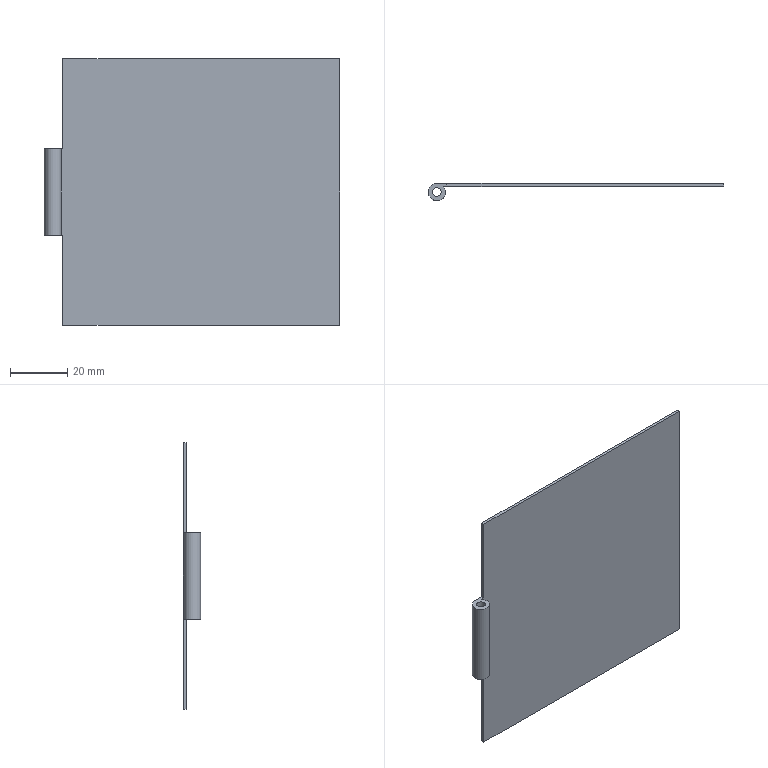Component | NX | PART_6 | 1 solid | 11 faces | box 103 x 6 x 93 mm | volume 9669 mm3 | plane 9 | cylinder 2 | commonest cylinder face diameters 6 x1 3 x1
STEP:
#1=CARTESIAN_POINT('',(0.,0.,0.));
#2=DIRECTION('',(0.,0.,1.));
#3=DIRECTION('',(1.,0.,0.));
#4=AXIS2_PLACEMENT_3D('',#1,#2,#3);
#5=CARTESIAN_POINT('',(-46.5,19.,65.));
#6=VERTEX_POINT('',#5);
#7=CARTESIAN_POINT('',(-46.5,19.,96.5));
#8=VERTEX_POINT('',#7);
#9=CARTESIAN_POINT('',(-46.5,19.,-0.));
#10=DIRECTION('',(0.,0.,1.));
#11=VECTOR('',#10,1.);
#12=LINE('',#9,#11);
#13=CARTESIAN_POINT('',(-50.,19.,-0.));
#14=DIRECTION('',(-0.,-1.,0.));
#15=DIRECTION('',(-1.,0.,0.));
#16=AXIS2_PLACEMENT_3D('',#13,#14,#15);
#17=PLANE('',#16);
#18=CARTESIAN_POINT('',(-3.5,0.));
#19=DIRECTION('',(0.,-1.));
#20=VECTOR('',#19,1.);
#21=LINE('',#18,#20);
#22=(GEOMETRIC_REPRESENTATION_CONTEXT(2)PARAMETRIC_REPRESENTATION_CONTEXT()REPRESENTATION_CONTEXT('',''));
#23=DEFINITIONAL_REPRESENTATION('',(#21),#22);
#24=PCURVE('',#17,#23);
#25=CARTESIAN_POINT('',(-46.5,18.5,82.75));
#26=DIRECTION('',(1.,0.,0.));
#27=DIRECTION('',(0.,0.,1.));
#28=AXIS2_PLACEMENT_3D('',#25,#26,#27);
#29=PLANE('',#28);
#30=CARTESIAN_POINT('',(-82.75,-0.5));
#31=DIRECTION('',(1.,0.));
#32=VECTOR('',#31,1.);
#33=LINE('',#30,#32);
#34=(GEOMETRIC_REPRESENTATION_CONTEXT(2)PARAMETRIC_REPRESENTATION_CONTEXT()REPRESENTATION_CONTEXT('',''));
#35=DEFINITIONAL_REPRESENTATION('',(#33),#34);
#36=PCURVE('',#29,#35);
#37=SURFACE_CURVE('',#12,(#24,#36),.PCURVE_S1.);
#38=EDGE_CURVE('',#6,#8,#37,.T.);
#39=ORIENTED_EDGE('',*,*,#38,.T.);
#40=CARTESIAN_POINT('',(50.,19.,96.5));
#41=VERTEX_POINT('',#40);
#42=CARTESIAN_POINT('',(-50.,19.,96.5));
#43=DIRECTION('',(1.,-0.,0.));
#44=VECTOR('',#43,1.);
#45=LINE('',#42,#44);
#46=CARTESIAN_POINT('',(0.,-96.5));
#47=DIRECTION('',(-1.,0.));
#48=VECTOR('',#47,1.);
#49=LINE('',#46,#48);
#50=(GEOMETRIC_REPRESENTATION_CONTEXT(2)PARAMETRIC_REPRESENTATION_CONTEXT()REPRESENTATION_CONTEXT('',''));
#51=DEFINITIONAL_REPRESENTATION('',(#49),#50);
#52=PCURVE('',#17,#51);
#53=CARTESIAN_POINT('',(50.5,18.5,96.5));
#54=DIRECTION('',(0.,0.,-1.));
#55=DIRECTION('',(1.,0.,0.));
#56=AXIS2_PLACEMENT_3D('',#53,#54,#55);
#57=PLANE('',#56);
#58=CARTESIAN_POINT('',(-100.5,-0.5));
#59=DIRECTION('',(1.,0.));
#60=VECTOR('',#59,1.);
#61=LINE('',#58,#60);
#62=(GEOMETRIC_REPRESENTATION_CONTEXT(2)PARAMETRIC_REPRESENTATION_CONTEXT()REPRESENTATION_CONTEXT('',''));
#63=DEFINITIONAL_REPRESENTATION('',(#61),#62);
#64=PCURVE('',#57,#63);
#65=SURFACE_CURVE('',#45,(#52,#64),.PCURVE_S1.);
#66=EDGE_CURVE('',#8,#41,#65,.T.);
#67=ORIENTED_EDGE('',*,*,#66,.T.);
#68=CARTESIAN_POINT('',(50.,19.,3.5));
#69=VERTEX_POINT('',#68);
#70=CARTESIAN_POINT('',(50.,19.,50.));
#71=DIRECTION('',(0.,0.,1.));
#72=VECTOR('',#71,1.);
#73=LINE('',#70,#72);
#74=CARTESIAN_POINT('',(-100.,-50.));
#75=DIRECTION('',(0.,-1.));
#76=VECTOR('',#75,1.);
#77=LINE('',#74,#76);
#78=(GEOMETRIC_REPRESENTATION_CONTEXT(2)PARAMETRIC_REPRESENTATION_CONTEXT()REPRESENTATION_CONTEXT('',''));
#79=DEFINITIONAL_REPRESENTATION('',(#77),#78);
#80=PCURVE('',#17,#79);
#81=CARTESIAN_POINT('',(50.,21.,50.));
#82=DIRECTION('',(-1.,0.,0.));
#83=DIRECTION('',(0.,-1.,0.));
#84=AXIS2_PLACEMENT_3D('',#81,#82,#83);
#85=PLANE('',#84);
#86=CARTESIAN_POINT('',(2.,0.));
#87=DIRECTION('',(0.,1.));
#88=VECTOR('',#87,1.);
#89=LINE('',#86,#88);
#90=(GEOMETRIC_REPRESENTATION_CONTEXT(2)PARAMETRIC_REPRESENTATION_CONTEXT()REPRESENTATION_CONTEXT('',''));
#91=DEFINITIONAL_REPRESENTATION('',(#89),#90);
#92=PCURVE('',#85,#91);
#93=SURFACE_CURVE('',#73,(#80,#92),.PCURVE_S1.);
#94=EDGE_CURVE('',#69,#41,#93,.T.);
#95=ORIENTED_EDGE('',*,*,#94,.F.);
#96=CARTESIAN_POINT('',(-46.5,19.,3.5));
#97=VERTEX_POINT('',#96);
#98=CARTESIAN_POINT('',(-50.,19.,3.5));
#99=DIRECTION('',(-1.,0.,0.));
#100=VECTOR('',#99,1.);
#101=LINE('',#98,#100);
#102=CARTESIAN_POINT('',(0.,-3.5));
#103=DIRECTION('',(1.,0.));
#104=VECTOR('',#103,1.);
#105=LINE('',#102,#104);
#106=(GEOMETRIC_REPRESENTATION_CONTEXT(2)PARAMETRIC_REPRESENTATION_CONTEXT()REPRESENTATION_CONTEXT('',''));
#107=DEFINITIONAL_REPRESENTATION('',(#105),#106);
#108=PCURVE('',#17,#107);
#109=CARTESIAN_POINT('',(50.5,18.5,3.5));
#110=DIRECTION('',(0.,0.,1.));
#111=DIRECTION('',(-1.,0.,0.));
#112=AXIS2_PLACEMENT_3D('',#109,#110,#111);
#113=PLANE('',#112);
#114=CARTESIAN_POINT('',(100.5,-0.5));
#115=DIRECTION('',(1.,-0.));
#116=VECTOR('',#115,1.);
#117=LINE('',#114,#116);
#118=(GEOMETRIC_REPRESENTATION_CONTEXT(2)PARAMETRIC_REPRESENTATION_CONTEXT()REPRESENTATION_CONTEXT('',''));
#119=DEFINITIONAL_REPRESENTATION('',(#117),#118);
#120=PCURVE('',#113,#119);
#121=SURFACE_CURVE('',#101,(#108,#120),.PCURVE_S1.);
#122=EDGE_CURVE('',#69,#97,#121,.T.);
#123=ORIENTED_EDGE('',*,*,#122,.T.);
#124=CARTESIAN_POINT('',(-46.5,19.,35.));
#125=VERTEX_POINT('',#124);
#126=CARTESIAN_POINT('',(-46.5,19.,-0.));
#127=DIRECTION('',(0.,0.,1.));
#128=VECTOR('',#127,1.);
#129=LINE('',#126,#128);
#130=CARTESIAN_POINT('',(-3.5,0.));
#131=DIRECTION('',(0.,-1.));
#132=VECTOR('',#131,1.);
#133=LINE('',#130,#132);
#134=(GEOMETRIC_REPRESENTATION_CONTEXT(2)PARAMETRIC_REPRESENTATION_CONTEXT()REPRESENTATION_CONTEXT('',''));
#135=DEFINITIONAL_REPRESENTATION('',(#133),#134);
#136=PCURVE('',#17,#135);
#137=CARTESIAN_POINT('',(-46.5,18.5,17.25));
#138=DIRECTION('',(1.,0.,0.));
#139=DIRECTION('',(0.,0.,1.));
#140=AXIS2_PLACEMENT_3D('',#137,#138,#139);
#141=PLANE('',#140);
#142=CARTESIAN_POINT('',(-17.25,-0.5));
#143=DIRECTION('',(1.,0.));
#144=VECTOR('',#143,1.);
#145=LINE('',#142,#144);
#146=(GEOMETRIC_REPRESENTATION_CONTEXT(2)PARAMETRIC_REPRESENTATION_CONTEXT()REPRESENTATION_CONTEXT('',''));
#147=DEFINITIONAL_REPRESENTATION('',(#145),#146);
#148=PCURVE('',#141,#147);
#149=SURFACE_CURVE('',#129,(#136,#148),.PCURVE_S1.);
#150=EDGE_CURVE('',#97,#125,#149,.T.);
#151=ORIENTED_EDGE('',*,*,#150,.T.);
#152=CARTESIAN_POINT('',(-50.,19.,35.));
#153=VERTEX_POINT('',#152);
#154=CARTESIAN_POINT('',(-50.,19.,35.));
#155=DIRECTION('',(-1.,0.,0.));
#156=VECTOR('',#155,1.);
#157=LINE('',#154,#156);
#158=CARTESIAN_POINT('',(0.,-35.));
#159=DIRECTION('',(1.,0.));
#160=VECTOR('',#159,1.);
#161=LINE('',#158,#160);
#162=(GEOMETRIC_REPRESENTATION_CONTEXT(2)PARAMETRIC_REPRESENTATION_CONTEXT()REPRESENTATION_CONTEXT('',''));
#163=DEFINITIONAL_REPRESENTATION('',(#161),#162);
#164=PCURVE('',#17,#163);
#165=CARTESIAN_POINT('',(-50.,16.,35.));
#166=DIRECTION('',(0.,0.,-1.));
#167=DIRECTION('',(1.,0.,0.));
#168=AXIS2_PLACEMENT_3D('',#165,#166,#167);
#169=PLANE('',#168);
#170=CARTESIAN_POINT('',(0.,-3.));
#171=DIRECTION('',(-1.,-0.));
#172=VECTOR('',#171,1.);
#173=LINE('',#170,#172);
#174=(GEOMETRIC_REPRESENTATION_CONTEXT(2)PARAMETRIC_REPRESENTATION_CONTEXT()REPRESENTATION_CONTEXT('',''));
#175=DEFINITIONAL_REPRESENTATION('',(#173),#174);
#176=PCURVE('',#169,#175);
#177=SURFACE_CURVE('',#157,(#164,#176),.PCURVE_S1.);
#178=EDGE_CURVE('',#125,#153,#177,.T.);
#179=ORIENTED_EDGE('',*,*,#178,.T.);
#180=CARTESIAN_POINT('',(-50.,19.,65.));
#181=VERTEX_POINT('',#180);
#182=CARTESIAN_POINT('',(-50.,19.,-0.));
#183=DIRECTION('',(0.,0.,1.));
#184=VECTOR('',#183,1.);
#185=LINE('',#182,#184);
#186=CARTESIAN_POINT('',(0.,0.));
#187=DIRECTION('',(0.,-1.));
#188=VECTOR('',#187,1.);
#189=LINE('',#186,#188);
#190=(GEOMETRIC_REPRESENTATION_CONTEXT(2)PARAMETRIC_REPRESENTATION_CONTEXT()REPRESENTATION_CONTEXT('',''));
#191=DEFINITIONAL_REPRESENTATION('',(#189),#190);
#192=PCURVE('',#17,#191);
#193=CARTESIAN_POINT('',(-50.,16.,35.));
#194=DIRECTION('',(0.,0.,1.));
#195=DIRECTION('',(-1.,0.,0.));
#196=AXIS2_PLACEMENT_3D('',#193,#194,#195);
#197=CYLINDRICAL_SURFACE('',#196,3.);
#198=CARTESIAN_POINT('',(-1.571,-35.));
#199=DIRECTION('',(0.,1.));
#200=VECTOR('',#199,1.);
#201=LINE('',#198,#200);
#202=(GEOMETRIC_REPRESENTATION_CONTEXT(2)PARAMETRIC_REPRESENTATION_CONTEXT()REPRESENTATION_CONTEXT('',''));
#203=DEFINITIONAL_REPRESENTATION('',(#201),#202);
#204=PCURVE('',#197,#203);
#205=SURFACE_CURVE('',#185,(#192,#204),.PCURVE_S1.);
#206=EDGE_CURVE('',#153,#181,#205,.T.);
#207=ORIENTED_EDGE('',*,*,#206,.T.);
#208=CARTESIAN_POINT('',(-50.,19.,65.));
#209=DIRECTION('',(1.,-0.,0.));
#210=VECTOR('',#209,1.);
#211=LINE('',#208,#210);
#212=CARTESIAN_POINT('',(0.,-65.));
#213=DIRECTION('',(-1.,0.));
#214=VECTOR('',#213,1.);
#215=LINE('',#212,#214);
#216=(GEOMETRIC_REPRESENTATION_CONTEXT(2)PARAMETRIC_REPRESENTATION_CONTEXT()REPRESENTATION_CONTEXT('',''));
#217=DEFINITIONAL_REPRESENTATION('',(#215),#216);
#218=PCURVE('',#17,#217);
#219=CARTESIAN_POINT('',(-50.,16.,65.));
#220=DIRECTION('',(0.,0.,-1.));
#221=DIRECTION('',(1.,0.,0.));
#222=AXIS2_PLACEMENT_3D('',#219,#220,#221);
#223=PLANE('',#222);
#224=CARTESIAN_POINT('',(0.,-3.));
#225=DIRECTION('',(1.,0.));
#226=VECTOR('',#225,1.);
#227=LINE('',#224,#226);
#228=(GEOMETRIC_REPRESENTATION_CONTEXT(2)PARAMETRIC_REPRESENTATION_CONTEXT()REPRESENTATION_CONTEXT('',''));
#229=DEFINITIONAL_REPRESENTATION('',(#227),#228);
#230=PCURVE('',#223,#229);
#231=SURFACE_CURVE('',#211,(#218,#230),.PCURVE_S1.);
#232=EDGE_CURVE('',#181,#6,#231,.T.);
#233=ORIENTED_EDGE('',*,*,#232,.T.);
#234=EDGE_LOOP('',(#39,#67,#95,#123,#151,#179,#207,#233));
#235=FACE_BOUND('',#234,.T.);
#236=ADVANCED_FACE('',(#235),#17,.F.);
#237=ORIENTED_EDGE('',*,*,#94,.T.);
#238=CARTESIAN_POINT('',(50.,18.,96.5));
#239=VERTEX_POINT('',#238);
#240=CARTESIAN_POINT('',(50.,21.,96.5));
#241=DIRECTION('',(0.,-1.,0.));
#242=VECTOR('',#241,1.);
#243=LINE('',#240,#242);
#244=CARTESIAN_POINT('',(0.,46.5));
#245=DIRECTION('',(1.,0.));
#246=VECTOR('',#245,1.);
#247=LINE('',#244,#246);
#248=(GEOMETRIC_REPRESENTATION_CONTEXT(2)PARAMETRIC_REPRESENTATION_CONTEXT()REPRESENTATION_CONTEXT('',''));
#249=DEFINITIONAL_REPRESENTATION('',(#247),#248);
#250=PCURVE('',#85,#249);
#251=CARTESIAN_POINT('',(-0.5,-2.5));
#252=DIRECTION('',(0.,1.));
#253=VECTOR('',#252,1.);
#254=LINE('',#251,#253);
#255=(GEOMETRIC_REPRESENTATION_CONTEXT(2)PARAMETRIC_REPRESENTATION_CONTEXT()REPRESENTATION_CONTEXT('',''));
#256=DEFINITIONAL_REPRESENTATION('',(#254),#255);
#257=PCURVE('',#57,#256);
#258=SURFACE_CURVE('',#243,(#250,#257),.PCURVE_S1.);
#259=EDGE_CURVE('',#41,#239,#258,.T.);
#260=ORIENTED_EDGE('',*,*,#259,.T.);
#261=CARTESIAN_POINT('',(50.,18.,3.5));
#262=VERTEX_POINT('',#261);
#263=CARTESIAN_POINT('',(50.,18.,-0.));
#264=DIRECTION('',(0.,0.,1.));
#265=VECTOR('',#264,1.);
#266=LINE('',#263,#265);
#267=CARTESIAN_POINT('',(3.,-50.));
#268=DIRECTION('',(0.,1.));
#269=VECTOR('',#268,1.);
#270=LINE('',#267,#269);
#271=(GEOMETRIC_REPRESENTATION_CONTEXT(2)PARAMETRIC_REPRESENTATION_CONTEXT()REPRESENTATION_CONTEXT('',''));
#272=DEFINITIONAL_REPRESENTATION('',(#270),#271);
#273=PCURVE('',#85,#272);
#274=CARTESIAN_POINT('',(50.,18.,-0.));
#275=DIRECTION('',(0.,1.,0.));
#276=DIRECTION('',(1.,-0.,0.));
#277=AXIS2_PLACEMENT_3D('',#274,#275,#276);
#278=PLANE('',#277);
#279=CARTESIAN_POINT('',(0.,0.));
#280=DIRECTION('',(0.,-1.));
#281=VECTOR('',#280,1.);
#282=LINE('',#279,#281);
#283=(GEOMETRIC_REPRESENTATION_CONTEXT(2)PARAMETRIC_REPRESENTATION_CONTEXT()REPRESENTATION_CONTEXT('',''));
#284=DEFINITIONAL_REPRESENTATION('',(#282),#283);
#285=PCURVE('',#278,#284);
#286=SURFACE_CURVE('',#266,(#273,#285),.PCURVE_S1.);
#287=EDGE_CURVE('',#262,#239,#286,.T.);
#288=ORIENTED_EDGE('',*,*,#287,.F.);
#289=CARTESIAN_POINT('',(50.,21.,3.5));
#290=DIRECTION('',(0.,1.,0.));
#291=VECTOR('',#290,1.);
#292=LINE('',#289,#291);
#293=CARTESIAN_POINT('',(0.,-46.5));
#294=DIRECTION('',(-1.,0.));
#295=VECTOR('',#294,1.);
#296=LINE('',#293,#295);
#297=(GEOMETRIC_REPRESENTATION_CONTEXT(2)PARAMETRIC_REPRESENTATION_CONTEXT()REPRESENTATION_CONTEXT('',''));
#298=DEFINITIONAL_REPRESENTATION('',(#296),#297);
#299=PCURVE('',#85,#298);
#300=CARTESIAN_POINT('',(0.5,-2.5));
#301=DIRECTION('',(0.,-1.));
#302=VECTOR('',#301,1.);
#303=LINE('',#300,#302);
#304=(GEOMETRIC_REPRESENTATION_CONTEXT(2)PARAMETRIC_REPRESENTATION_CONTEXT()REPRESENTATION_CONTEXT('',''));
#305=DEFINITIONAL_REPRESENTATION('',(#303),#304);
#306=PCURVE('',#113,#305);
#307=SURFACE_CURVE('',#292,(#299,#306),.PCURVE_S1.);
#308=EDGE_CURVE('',#262,#69,#307,.T.);
#309=ORIENTED_EDGE('',*,*,#308,.T.);
#310=EDGE_LOOP('',(#237,#260,#288,#309));
#311=FACE_BOUND('',#310,.T.);
#312=ADVANCED_FACE('',(#311),#85,.F.);
#313=ORIENTED_EDGE('',*,*,#287,.T.);
#314=CARTESIAN_POINT('',(-46.5,18.,96.5));
#315=VERTEX_POINT('',#314);
#316=CARTESIAN_POINT('',(50.,18.,96.5));
#317=DIRECTION('',(-1.,0.,0.));
#318=VECTOR('',#317,1.);
#319=LINE('',#316,#318);
#320=CARTESIAN_POINT('',(0.,-96.5));
#321=DIRECTION('',(-1.,0.));
#322=VECTOR('',#321,1.);
#323=LINE('',#320,#322);
#324=(GEOMETRIC_REPRESENTATION_CONTEXT(2)PARAMETRIC_REPRESENTATION_CONTEXT()REPRESENTATION_CONTEXT('',''));
#325=DEFINITIONAL_REPRESENTATION('',(#323),#324);
#326=PCURVE('',#278,#325);
#327=CARTESIAN_POINT('',(-0.5,0.5));
#328=DIRECTION('',(-1.,-0.));
#329=VECTOR('',#328,1.);
#330=LINE('',#327,#329);
#331=(GEOMETRIC_REPRESENTATION_CONTEXT(2)PARAMETRIC_REPRESENTATION_CONTEXT()REPRESENTATION_CONTEXT('',''));
#332=DEFINITIONAL_REPRESENTATION('',(#330),#331);
#333=PCURVE('',#57,#332);
#334=SURFACE_CURVE('',#319,(#326,#333),.PCURVE_S1.);
#335=EDGE_CURVE('',#239,#315,#334,.T.);
#336=ORIENTED_EDGE('',*,*,#335,.T.);
#337=CARTESIAN_POINT('',(-46.5,18.,65.));
#338=VERTEX_POINT('',#337);
#339=CARTESIAN_POINT('',(-46.5,18.,-0.));
#340=DIRECTION('',(0.,0.,-1.));
#341=VECTOR('',#340,1.);
#342=LINE('',#339,#341);
#343=CARTESIAN_POINT('',(-96.5,0.));
#344=DIRECTION('',(0.,1.));
#345=VECTOR('',#344,1.);
#346=LINE('',#343,#345);
#347=(GEOMETRIC_REPRESENTATION_CONTEXT(2)PARAMETRIC_REPRESENTATION_CONTEXT()REPRESENTATION_CONTEXT('',''));
#348=DEFINITIONAL_REPRESENTATION('',(#346),#347);
#349=PCURVE('',#278,#348);
#350=CARTESIAN_POINT('',(-82.75,0.5));
#351=DIRECTION('',(-1.,0.));
#352=VECTOR('',#351,1.);
#353=LINE('',#350,#352);
#354=(GEOMETRIC_REPRESENTATION_CONTEXT(2)PARAMETRIC_REPRESENTATION_CONTEXT()REPRESENTATION_CONTEXT('',''));
#355=DEFINITIONAL_REPRESENTATION('',(#353),#354);
#356=PCURVE('',#29,#355);
#357=SURFACE_CURVE('',#342,(#349,#356),.PCURVE_S1.);
#358=EDGE_CURVE('',#315,#338,#357,.T.);
#359=ORIENTED_EDGE('',*,*,#358,.T.);
#360=CARTESIAN_POINT('',(-47.764,18.,65.));
#361=VERTEX_POINT('',#360);
#362=CARTESIAN_POINT('',(50.,18.,65.));
#363=DIRECTION('',(1.,-0.,0.));
#364=VECTOR('',#363,1.);
#365=LINE('',#362,#364);
#366=CARTESIAN_POINT('',(0.,-65.));
#367=DIRECTION('',(1.,0.));
#368=VECTOR('',#367,1.);
#369=LINE('',#366,#368);
#370=(GEOMETRIC_REPRESENTATION_CONTEXT(2)PARAMETRIC_REPRESENTATION_CONTEXT()REPRESENTATION_CONTEXT('',''));
#371=DEFINITIONAL_REPRESENTATION('',(#369),#370);
#372=PCURVE('',#278,#371);
#373=CARTESIAN_POINT('',(100.,-2.));
#374=DIRECTION('',(1.,0.));
#375=VECTOR('',#374,1.);
#376=LINE('',#373,#375);
#377=(GEOMETRIC_REPRESENTATION_CONTEXT(2)PARAMETRIC_REPRESENTATION_CONTEXT()REPRESENTATION_CONTEXT('',''));
#378=DEFINITIONAL_REPRESENTATION('',(#376),#377);
#379=PCURVE('',#223,#378);
#380=SURFACE_CURVE('',#365,(#372,#379),.PCURVE_S1.);
#381=EDGE_CURVE('',#361,#338,#380,.T.);
#382=ORIENTED_EDGE('',*,*,#381,.F.);
#383=CARTESIAN_POINT('',(-47.764,18.,35.));
#384=VERTEX_POINT('',#383);
#385=CARTESIAN_POINT('',(-47.764,18.,35.));
#386=DIRECTION('',(0.,0.,1.));
#387=VECTOR('',#386,1.);
#388=LINE('',#385,#387);
#389=CARTESIAN_POINT('',(-97.764,-35.));
#390=DIRECTION('',(0.,-1.));
#391=VECTOR('',#390,1.);
#392=LINE('',#389,#391);
#393=(GEOMETRIC_REPRESENTATION_CONTEXT(2)PARAMETRIC_REPRESENTATION_CONTEXT()REPRESENTATION_CONTEXT('',''));
#394=DEFINITIONAL_REPRESENTATION('',(#392),#393);
#395=PCURVE('',#278,#394);
#396=CARTESIAN_POINT('',(3.871,0.));
#397=DIRECTION('',(0.,1.));
#398=VECTOR('',#397,1.);
#399=LINE('',#396,#398);
#400=(GEOMETRIC_REPRESENTATION_CONTEXT(2)PARAMETRIC_REPRESENTATION_CONTEXT()REPRESENTATION_CONTEXT('',''));
#401=DEFINITIONAL_REPRESENTATION('',(#399),#400);
#402=PCURVE('',#197,#401);
#403=SURFACE_CURVE('',#388,(#395,#402),.PCURVE_S1.);
#404=EDGE_CURVE('',#384,#361,#403,.T.);
#405=ORIENTED_EDGE('',*,*,#404,.F.);
#406=CARTESIAN_POINT('',(-46.5,18.,35.));
#407=VERTEX_POINT('',#406);
#408=CARTESIAN_POINT('',(50.,18.,35.));
#409=DIRECTION('',(1.,-0.,0.));
#410=VECTOR('',#409,1.);
#411=LINE('',#408,#410);
#412=CARTESIAN_POINT('',(0.,-35.));
#413=DIRECTION('',(1.,0.));
#414=VECTOR('',#413,1.);
#415=LINE('',#412,#414);
#416=(GEOMETRIC_REPRESENTATION_CONTEXT(2)PARAMETRIC_REPRESENTATION_CONTEXT()REPRESENTATION_CONTEXT('',''));
#417=DEFINITIONAL_REPRESENTATION('',(#415),#416);
#418=PCURVE('',#278,#417);
#419=CARTESIAN_POINT('',(100.,-2.));
#420=DIRECTION('',(1.,0.));
#421=VECTOR('',#420,1.);
#422=LINE('',#419,#421);
#423=(GEOMETRIC_REPRESENTATION_CONTEXT(2)PARAMETRIC_REPRESENTATION_CONTEXT()REPRESENTATION_CONTEXT('',''));
#424=DEFINITIONAL_REPRESENTATION('',(#422),#423);
#425=PCURVE('',#169,#424);
#426=SURFACE_CURVE('',#411,(#418,#425),.PCURVE_S1.);
#427=EDGE_CURVE('',#384,#407,#426,.T.);
#428=ORIENTED_EDGE('',*,*,#427,.T.);
#429=CARTESIAN_POINT('',(-46.5,18.,3.5));
#430=VERTEX_POINT('',#429);
#431=CARTESIAN_POINT('',(-46.5,18.,-0.));
#432=DIRECTION('',(0.,0.,-1.));
#433=VECTOR('',#432,1.);
#434=LINE('',#431,#433);
#435=CARTESIAN_POINT('',(-96.5,0.));
#436=DIRECTION('',(0.,1.));
#437=VECTOR('',#436,1.);
#438=LINE('',#435,#437);
#439=(GEOMETRIC_REPRESENTATION_CONTEXT(2)PARAMETRIC_REPRESENTATION_CONTEXT()REPRESENTATION_CONTEXT('',''));
#440=DEFINITIONAL_REPRESENTATION('',(#438),#439);
#441=PCURVE('',#278,#440);
#442=CARTESIAN_POINT('',(-17.25,0.5));
#443=DIRECTION('',(-1.,0.));
#444=VECTOR('',#443,1.);
#445=LINE('',#442,#444);
#446=(GEOMETRIC_REPRESENTATION_CONTEXT(2)PARAMETRIC_REPRESENTATION_CONTEXT()REPRESENTATION_CONTEXT('',''));
#447=DEFINITIONAL_REPRESENTATION('',(#445),#446);
#448=PCURVE('',#141,#447);
#449=SURFACE_CURVE('',#434,(#441,#448),.PCURVE_S1.);
#450=EDGE_CURVE('',#407,#430,#449,.T.);
#451=ORIENTED_EDGE('',*,*,#450,.T.);
#452=CARTESIAN_POINT('',(50.,18.,3.5));
#453=DIRECTION('',(1.,-0.,0.));
#454=VECTOR('',#453,1.);
#455=LINE('',#452,#454);
#456=CARTESIAN_POINT('',(0.,-3.5));
#457=DIRECTION('',(1.,0.));
#458=VECTOR('',#457,1.);
#459=LINE('',#456,#458);
#460=(GEOMETRIC_REPRESENTATION_CONTEXT(2)PARAMETRIC_REPRESENTATION_CONTEXT()REPRESENTATION_CONTEXT('',''));
#461=DEFINITIONAL_REPRESENTATION('',(#459),#460);
#462=PCURVE('',#278,#461);
#463=CARTESIAN_POINT('',(0.5,0.5));
#464=DIRECTION('',(-1.,0.));
#465=VECTOR('',#464,1.);
#466=LINE('',#463,#465);
#467=(GEOMETRIC_REPRESENTATION_CONTEXT(2)PARAMETRIC_REPRESENTATION_CONTEXT()REPRESENTATION_CONTEXT('',''));
#468=DEFINITIONAL_REPRESENTATION('',(#466),#467);
#469=PCURVE('',#113,#468);
#470=SURFACE_CURVE('',#455,(#462,#469),.PCURVE_S1.);
#471=EDGE_CURVE('',#430,#262,#470,.T.);
#472=ORIENTED_EDGE('',*,*,#471,.T.);
#473=EDGE_LOOP('',(#313,#336,#359,#382,#405,#428,#451,#472));
#474=FACE_BOUND('',#473,.T.);
#475=ADVANCED_FACE('',(#474),#278,.F.);
#476=CARTESIAN_POINT('',(-50.,16.,35.));
#477=DIRECTION('',(0.,0.,-1.));
#478=DIRECTION('',(0.,-1.,0.));
#479=AXIS2_PLACEMENT_3D('',#476,#477,#478);
#480=CIRCLE('',#479,3.);
#481=CARTESIAN_POINT('',(7.854,0.));
#482=DIRECTION('',(-1.,0.));
#483=VECTOR('',#482,1.);
#484=LINE('',#481,#483);
#485=(GEOMETRIC_REPRESENTATION_CONTEXT(2)PARAMETRIC_REPRESENTATION_CONTEXT()REPRESENTATION_CONTEXT('',''));
#486=DEFINITIONAL_REPRESENTATION('',(#484),#485);
#487=PCURVE('',#197,#486);
#488=CARTESIAN_POINT('',(0.,0.));
#489=DIRECTION('',(0.,1.));
#490=AXIS2_PLACEMENT_2D('',#488,#489);
#491=CIRCLE('',#490,3.);
#492=(GEOMETRIC_REPRESENTATION_CONTEXT(2)PARAMETRIC_REPRESENTATION_CONTEXT()REPRESENTATION_CONTEXT('',''));
#493=DEFINITIONAL_REPRESENTATION('',(#491),#492);
#494=PCURVE('',#169,#493);
#495=SURFACE_CURVE('',#480,(#487,#494),.PCURVE_S1.);
#496=EDGE_CURVE('',#384,#153,#495,.T.);
#497=ORIENTED_EDGE('',*,*,#496,.F.);
#498=ORIENTED_EDGE('',*,*,#404,.T.);
#499=CARTESIAN_POINT('',(-50.,16.,65.));
#500=DIRECTION('',(0.,0.,-1.));
#501=DIRECTION('',(0.,-1.,0.));
#502=AXIS2_PLACEMENT_3D('',#499,#500,#501);
#503=CIRCLE('',#502,3.);
#504=CARTESIAN_POINT('',(7.854,30.));
#505=DIRECTION('',(-1.,0.));
#506=VECTOR('',#505,1.);
#507=LINE('',#504,#506);
#508=(GEOMETRIC_REPRESENTATION_CONTEXT(2)PARAMETRIC_REPRESENTATION_CONTEXT()REPRESENTATION_CONTEXT('',''));
#509=DEFINITIONAL_REPRESENTATION('',(#507),#508);
#510=PCURVE('',#197,#509);
#511=CARTESIAN_POINT('',(0.,0.));
#512=DIRECTION('',(0.,1.));
#513=AXIS2_PLACEMENT_2D('',#511,#512);
#514=CIRCLE('',#513,3.);
#515=(GEOMETRIC_REPRESENTATION_CONTEXT(2)PARAMETRIC_REPRESENTATION_CONTEXT()REPRESENTATION_CONTEXT('',''));
#516=DEFINITIONAL_REPRESENTATION('',(#514),#515);
#517=PCURVE('',#223,#516);
#518=SURFACE_CURVE('',#503,(#510,#517),.PCURVE_S1.);
#519=EDGE_CURVE('',#361,#181,#518,.T.);
#520=ORIENTED_EDGE('',*,*,#519,.T.);
#521=ORIENTED_EDGE('',*,*,#206,.F.);
#522=EDGE_LOOP('',(#497,#498,#520,#521));
#523=FACE_BOUND('',#522,.T.);
#524=ADVANCED_FACE('',(#523),#197,.T.);
#525=CARTESIAN_POINT('',(-50.,14.5,35.));
#526=VERTEX_POINT('',#525);
#527=CARTESIAN_POINT('',(-50.,16.,35.));
#528=DIRECTION('',(0.,0.,-1.));
#529=DIRECTION('',(0.,-1.,0.));
#530=AXIS2_PLACEMENT_3D('',#527,#528,#529);
#531=CIRCLE('',#530,1.5);
#532=CARTESIAN_POINT('',(0.,0.));
#533=DIRECTION('',(0.,1.));
#534=AXIS2_PLACEMENT_2D('',#532,#533);
#535=CIRCLE('',#534,1.5);
#536=(GEOMETRIC_REPRESENTATION_CONTEXT(2)PARAMETRIC_REPRESENTATION_CONTEXT()REPRESENTATION_CONTEXT('',''));
#537=DEFINITIONAL_REPRESENTATION('',(#535),#536);
#538=PCURVE('',#169,#537);
#539=CARTESIAN_POINT('',(-50.,16.,35.));
#540=DIRECTION('',(0.,0.,1.));
#541=DIRECTION('',(-1.,0.,0.));
#542=AXIS2_PLACEMENT_3D('',#539,#540,#541);
#543=CYLINDRICAL_SURFACE('',#542,1.5);
#544=CARTESIAN_POINT('',(7.854,0.));
#545=DIRECTION('',(-1.,0.));
#546=VECTOR('',#545,1.);
#547=LINE('',#544,#546);
#548=(GEOMETRIC_REPRESENTATION_CONTEXT(2)PARAMETRIC_REPRESENTATION_CONTEXT()REPRESENTATION_CONTEXT('',''));
#549=DEFINITIONAL_REPRESENTATION('',(#547),#548);
#550=PCURVE('',#543,#549);
#551=SURFACE_CURVE('',#531,(#538,#550),.PCURVE_S1.);
#552=EDGE_CURVE('',#526,#526,#551,.T.);
#553=ORIENTED_EDGE('',*,*,#552,.F.);
#554=EDGE_LOOP('',(#553));
#555=FACE_BOUND('',#554,.T.);
#556=ORIENTED_EDGE('',*,*,#496,.T.);
#557=ORIENTED_EDGE('',*,*,#178,.F.);
#558=CARTESIAN_POINT('',(-46.5,18.5,35.));
#559=DIRECTION('',(0.,1.,0.));
#560=VECTOR('',#559,1.);
#561=LINE('',#558,#560);
#562=CARTESIAN_POINT('',(3.5,-2.5));
#563=DIRECTION('',(0.,-1.));
#564=VECTOR('',#563,1.);
#565=LINE('',#562,#564);
#566=(GEOMETRIC_REPRESENTATION_CONTEXT(2)PARAMETRIC_REPRESENTATION_CONTEXT()REPRESENTATION_CONTEXT('',''));
#567=DEFINITIONAL_REPRESENTATION('',(#565),#566);
#568=PCURVE('',#169,#567);
#569=CARTESIAN_POINT('',(17.75,0.));
#570=DIRECTION('',(0.,-1.));
#571=VECTOR('',#570,1.);
#572=LINE('',#569,#571);
#573=(GEOMETRIC_REPRESENTATION_CONTEXT(2)PARAMETRIC_REPRESENTATION_CONTEXT()REPRESENTATION_CONTEXT('',''));
#574=DEFINITIONAL_REPRESENTATION('',(#572),#573);
#575=PCURVE('',#141,#574);
#576=SURFACE_CURVE('',#561,(#568,#575),.PCURVE_S1.);
#577=EDGE_CURVE('',#407,#125,#576,.T.);
#578=ORIENTED_EDGE('',*,*,#577,.F.);
#579=ORIENTED_EDGE('',*,*,#427,.F.);
#580=EDGE_LOOP('',(#556,#557,#578,#579));
#581=FACE_BOUND('',#580,.T.);
#582=ADVANCED_FACE('',(#555,#581),#169,.T.);
#583=CARTESIAN_POINT('',(-50.,14.5,65.));
#584=VERTEX_POINT('',#583);
#585=CARTESIAN_POINT('',(-50.,16.,65.));
#586=DIRECTION('',(0.,0.,-1.));
#587=DIRECTION('',(0.,-1.,0.));
#588=AXIS2_PLACEMENT_3D('',#585,#586,#587);
#589=CIRCLE('',#588,1.5);
#590=CARTESIAN_POINT('',(0.,0.));
#591=DIRECTION('',(0.,1.));
#592=AXIS2_PLACEMENT_2D('',#590,#591);
#593=CIRCLE('',#592,1.5);
#594=(GEOMETRIC_REPRESENTATION_CONTEXT(2)PARAMETRIC_REPRESENTATION_CONTEXT()REPRESENTATION_CONTEXT('',''));
#595=DEFINITIONAL_REPRESENTATION('',(#593),#594);
#596=PCURVE('',#223,#595);
#597=CARTESIAN_POINT('',(7.854,30.));
#598=DIRECTION('',(-1.,0.));
#599=VECTOR('',#598,1.);
#600=LINE('',#597,#599);
#601=(GEOMETRIC_REPRESENTATION_CONTEXT(2)PARAMETRIC_REPRESENTATION_CONTEXT()REPRESENTATION_CONTEXT('',''));
#602=DEFINITIONAL_REPRESENTATION('',(#600),#601);
#603=PCURVE('',#543,#602);
#604=SURFACE_CURVE('',#589,(#596,#603),.PCURVE_S1.);
#605=EDGE_CURVE('',#584,#584,#604,.T.);
#606=ORIENTED_EDGE('',*,*,#605,.T.);
#607=EDGE_LOOP('',(#606));
#608=FACE_BOUND('',#607,.T.);
#609=ORIENTED_EDGE('',*,*,#232,.F.);
#610=ORIENTED_EDGE('',*,*,#519,.F.);
#611=ORIENTED_EDGE('',*,*,#381,.T.);
#612=CARTESIAN_POINT('',(-46.5,18.5,65.));
#613=DIRECTION('',(0.,-1.,0.));
#614=VECTOR('',#613,1.);
#615=LINE('',#612,#614);
#616=CARTESIAN_POINT('',(3.5,-2.5));
#617=DIRECTION('',(0.,1.));
#618=VECTOR('',#617,1.);
#619=LINE('',#616,#618);
#620=(GEOMETRIC_REPRESENTATION_CONTEXT(2)PARAMETRIC_REPRESENTATION_CONTEXT()REPRESENTATION_CONTEXT('',''));
#621=DEFINITIONAL_REPRESENTATION('',(#619),#620);
#622=PCURVE('',#223,#621);
#623=CARTESIAN_POINT('',(-17.75,0.));
#624=DIRECTION('',(0.,1.));
#625=VECTOR('',#624,1.);
#626=LINE('',#623,#625);
#627=(GEOMETRIC_REPRESENTATION_CONTEXT(2)PARAMETRIC_REPRESENTATION_CONTEXT()REPRESENTATION_CONTEXT('',''));
#628=DEFINITIONAL_REPRESENTATION('',(#626),#627);
#629=PCURVE('',#29,#628);
#630=SURFACE_CURVE('',#615,(#622,#629),.PCURVE_S1.);
#631=EDGE_CURVE('',#6,#338,#630,.T.);
#632=ORIENTED_EDGE('',*,*,#631,.F.);
#633=EDGE_LOOP('',(#609,#610,#611,#632));
#634=FACE_BOUND('',#633,.T.);
#635=ADVANCED_FACE('',(#608,#634),#223,.F.);
#636=ORIENTED_EDGE('',*,*,#552,.F.);
#637=CARTESIAN_POINT('',(-50.,14.5,35.));
#638=CARTESIAN_POINT('',(-50.,14.5,65.));
#639=B_SPLINE_CURVE_WITH_KNOTS('',1,(#637,#638),.UNSPECIFIED.,.F.,.F.,(2,2),(0.,30.),.PIECEWISE_BEZIER_KNOTS.);
#640=CARTESIAN_POINT('',(7.854,0.));
#641=DIRECTION('',(0.,1.));
#642=VECTOR('',#641,1.);
#643=LINE('',#640,#642);
#644=(GEOMETRIC_REPRESENTATION_CONTEXT(2)PARAMETRIC_REPRESENTATION_CONTEXT()REPRESENTATION_CONTEXT('',''));
#645=DEFINITIONAL_REPRESENTATION('',(#643),#644);
#646=PCURVE('',#543,#645);
#647=CARTESIAN_POINT('',(1.571,0.));
#648=DIRECTION('',(0.,1.));
#649=VECTOR('',#648,1.);
#650=LINE('',#647,#649);
#651=(GEOMETRIC_REPRESENTATION_CONTEXT(2)PARAMETRIC_REPRESENTATION_CONTEXT()REPRESENTATION_CONTEXT('',''));
#652=DEFINITIONAL_REPRESENTATION('',(#650),#651);
#653=PCURVE('',#543,#652);
#654=SEAM_CURVE('',#639,(#646,#653),.PCURVE_S1.);
#655=EDGE_CURVE('',#526,#584,#654,.T.);
#656=ORIENTED_EDGE('',*,*,#655,.T.);
#657=ORIENTED_EDGE('',*,*,#605,.T.);
#658=ORIENTED_EDGE('',*,*,#655,.F.);
#659=EDGE_LOOP('',(#636,#656,#657,#658));
#660=FACE_BOUND('',#659,.F.);
#661=ADVANCED_FACE('',(#660),#543,.F.);
#662=ORIENTED_EDGE('',*,*,#150,.F.);
#663=CARTESIAN_POINT('',(-46.5,18.5,3.5));
#664=DIRECTION('',(0.,-1.,0.));
#665=VECTOR('',#664,1.);
#666=LINE('',#663,#665);
#667=CARTESIAN_POINT('',(-13.75,0.));
#668=DIRECTION('',(0.,1.));
#669=VECTOR('',#668,1.);
#670=LINE('',#667,#669);
#671=(GEOMETRIC_REPRESENTATION_CONTEXT(2)PARAMETRIC_REPRESENTATION_CONTEXT()REPRESENTATION_CONTEXT('',''));
#672=DEFINITIONAL_REPRESENTATION('',(#670),#671);
#673=PCURVE('',#141,#672);
#674=CARTESIAN_POINT('',(97.,0.));
#675=DIRECTION('',(0.,1.));
#676=VECTOR('',#675,1.);
#677=LINE('',#674,#676);
#678=(GEOMETRIC_REPRESENTATION_CONTEXT(2)PARAMETRIC_REPRESENTATION_CONTEXT()REPRESENTATION_CONTEXT('',''));
#679=DEFINITIONAL_REPRESENTATION('',(#677),#678);
#680=PCURVE('',#113,#679);
#681=SURFACE_CURVE('',#666,(#673,#680),.PCURVE_S1.);
#682=EDGE_CURVE('',#97,#430,#681,.T.);
#683=ORIENTED_EDGE('',*,*,#682,.T.);
#684=ORIENTED_EDGE('',*,*,#450,.F.);
#685=ORIENTED_EDGE('',*,*,#577,.T.);
#686=EDGE_LOOP('',(#662,#683,#684,#685));
#687=FACE_BOUND('',#686,.T.);
#688=ADVANCED_FACE('',(#687),#141,.F.);
#689=ORIENTED_EDGE('',*,*,#358,.F.);
#690=CARTESIAN_POINT('',(-46.5,18.5,96.5));
#691=DIRECTION('',(0.,1.,0.));
#692=VECTOR('',#691,1.);
#693=LINE('',#690,#692);
#694=CARTESIAN_POINT('',(13.75,0.));
#695=DIRECTION('',(0.,-1.));
#696=VECTOR('',#695,1.);
#697=LINE('',#694,#696);
#698=(GEOMETRIC_REPRESENTATION_CONTEXT(2)PARAMETRIC_REPRESENTATION_CONTEXT()REPRESENTATION_CONTEXT('',''));
#699=DEFINITIONAL_REPRESENTATION('',(#697),#698);
#700=PCURVE('',#29,#699);
#701=CARTESIAN_POINT('',(-97.,0.));
#702=DIRECTION('',(0.,-1.));
#703=VECTOR('',#702,1.);
#704=LINE('',#701,#703);
#705=(GEOMETRIC_REPRESENTATION_CONTEXT(2)PARAMETRIC_REPRESENTATION_CONTEXT()REPRESENTATION_CONTEXT('',''));
#706=DEFINITIONAL_REPRESENTATION('',(#704),#705);
#707=PCURVE('',#57,#706);
#708=SURFACE_CURVE('',#693,(#700,#707),.PCURVE_S1.);
#709=EDGE_CURVE('',#315,#8,#708,.T.);
#710=ORIENTED_EDGE('',*,*,#709,.T.);
#711=ORIENTED_EDGE('',*,*,#38,.F.);
#712=ORIENTED_EDGE('',*,*,#631,.T.);
#713=EDGE_LOOP('',(#689,#710,#711,#712));
#714=FACE_BOUND('',#713,.T.);
#715=ADVANCED_FACE('',(#714),#29,.F.);
#716=ORIENTED_EDGE('',*,*,#308,.F.);
#717=ORIENTED_EDGE('',*,*,#471,.F.);
#718=ORIENTED_EDGE('',*,*,#682,.F.);
#719=ORIENTED_EDGE('',*,*,#122,.F.);
#720=EDGE_LOOP('',(#716,#717,#718,#719));
#721=FACE_BOUND('',#720,.T.);
#722=ADVANCED_FACE('',(#721),#113,.F.);
#723=ORIENTED_EDGE('',*,*,#709,.F.);
#724=ORIENTED_EDGE('',*,*,#335,.F.);
#725=ORIENTED_EDGE('',*,*,#259,.F.);
#726=ORIENTED_EDGE('',*,*,#66,.F.);
#727=EDGE_LOOP('',(#723,#724,#725,#726));
#728=FACE_BOUND('',#727,.T.);
#729=ADVANCED_FACE('',(#728),#57,.F.);
#730=CLOSED_SHELL('',(#236,#312,#475,#524,#582,#635,#661,#688,#715,#722,#729));
#731=MANIFOLD_SOLID_BREP('',#730);
#732=(LENGTH_UNIT()NAMED_UNIT(*)SI_UNIT(.MILLI.,.METRE.));
#733=UNCERTAINTY_MEASURE_WITH_UNIT(LENGTH_MEASURE(0.000001),#732,'','');
#734=(NAMED_UNIT(*)PLANE_ANGLE_UNIT()SI_UNIT($,.RADIAN.));
#735=(NAMED_UNIT(*)SI_UNIT($,.STERADIAN.)SOLID_ANGLE_UNIT());
#736=(GEOMETRIC_REPRESENTATION_CONTEXT(3)GLOBAL_UNCERTAINTY_ASSIGNED_CONTEXT((#733))GLOBAL_UNIT_ASSIGNED_CONTEXT((#732,#734,#735))REPRESENTATION_CONTEXT('',''));
#737=ADVANCED_BREP_SHAPE_REPRESENTATION('',(#4,#731),#736);